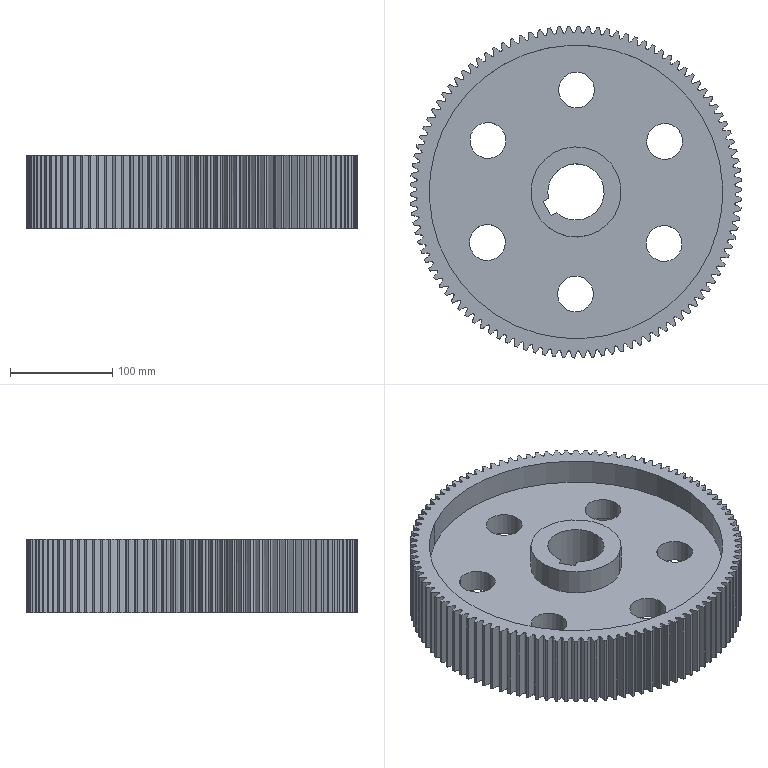Component | SolidWorks | CylindricalGear106_3-1 | 1 solid | 457 faces | volume 2482725 mm3 | cylinder 236 | spline 212 | plane 9 | commonest cylinder face diameters 324 x107 310.492 x106 35 x12 88 x4 286.5 x4 55 x3